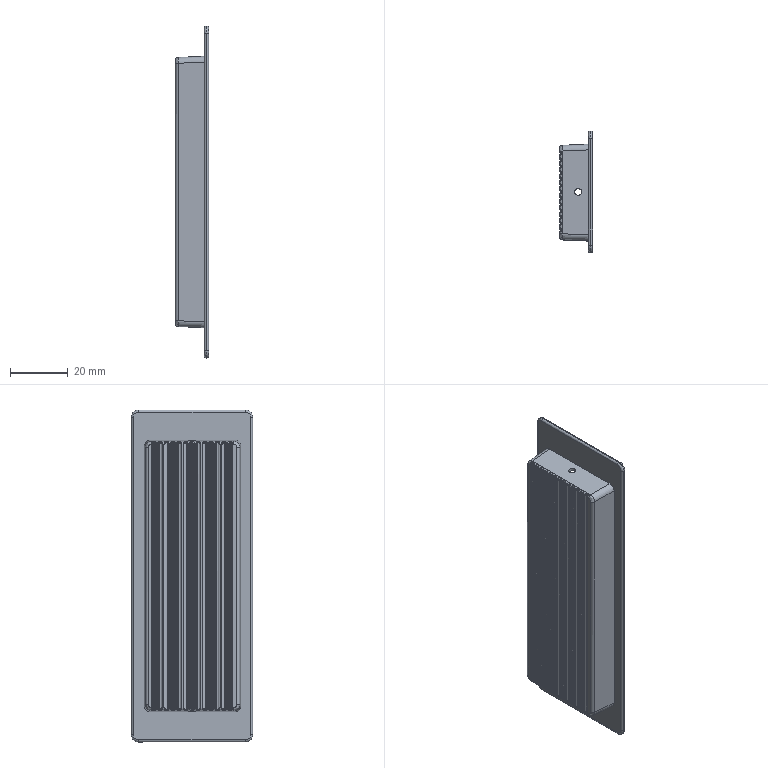Component | SolidWorks | PC-CAJ-P09-1_MANIJA  DE INCRUSTAR 115X40mm ACERO-1 | 2 solids | 293 faces | volume 9621 mm3 | cylinder 100 | plane 99 | spline 82 | torus 12 | commonest cylinder face diameters 1 x39 3 x25 1.4 x12 5 x8 2 x8 2.5 x4 4 x4 | material Plain Carbon Steel